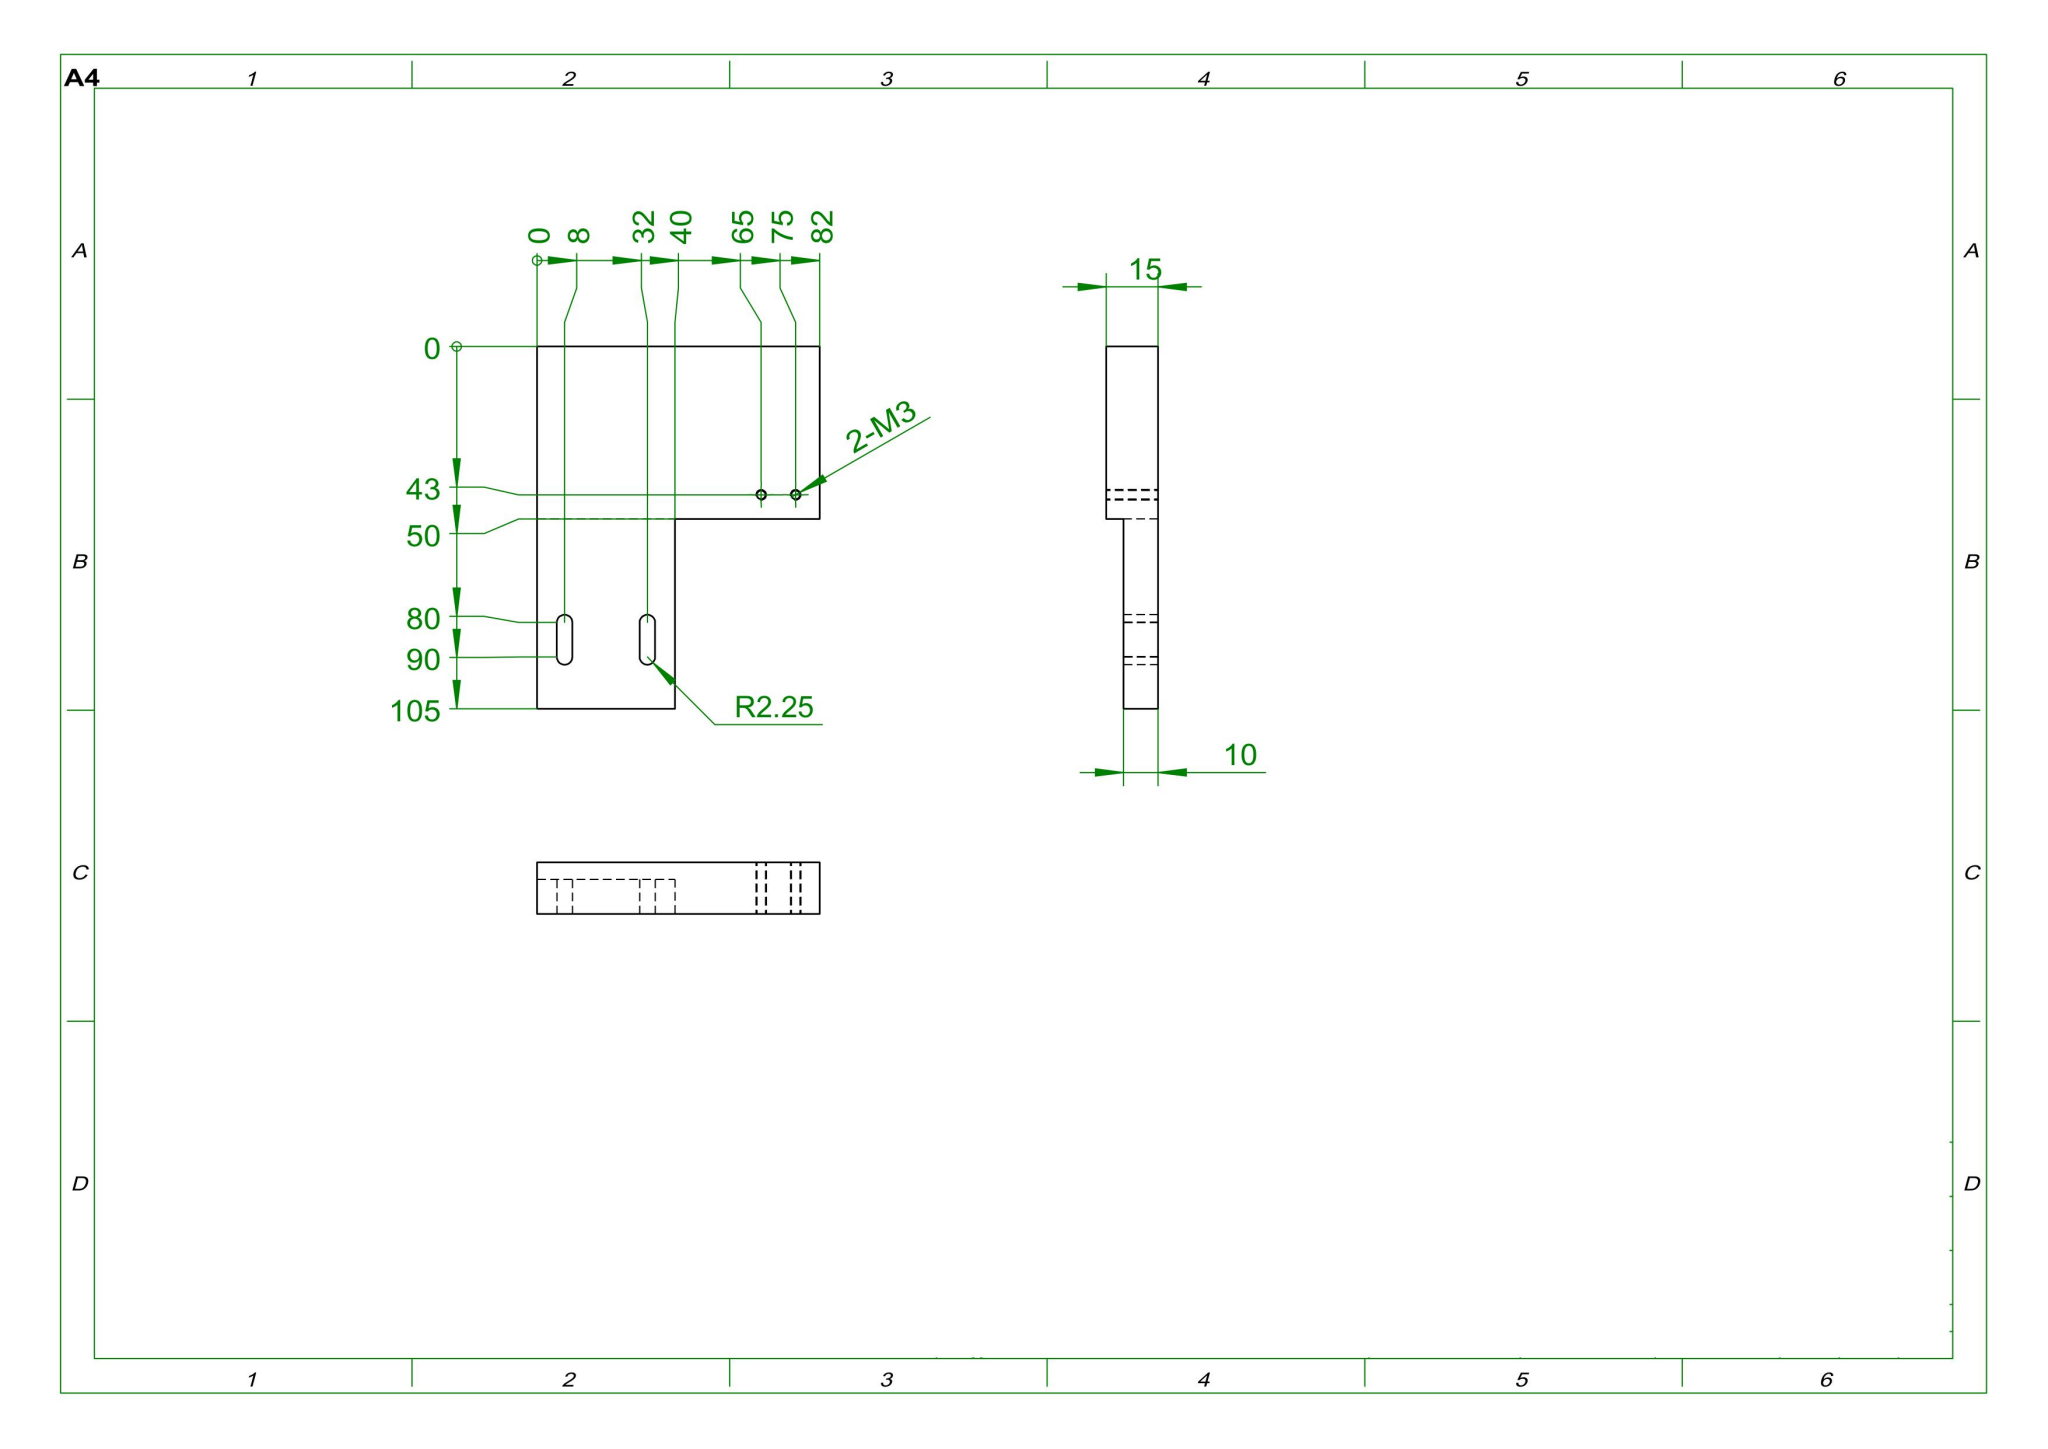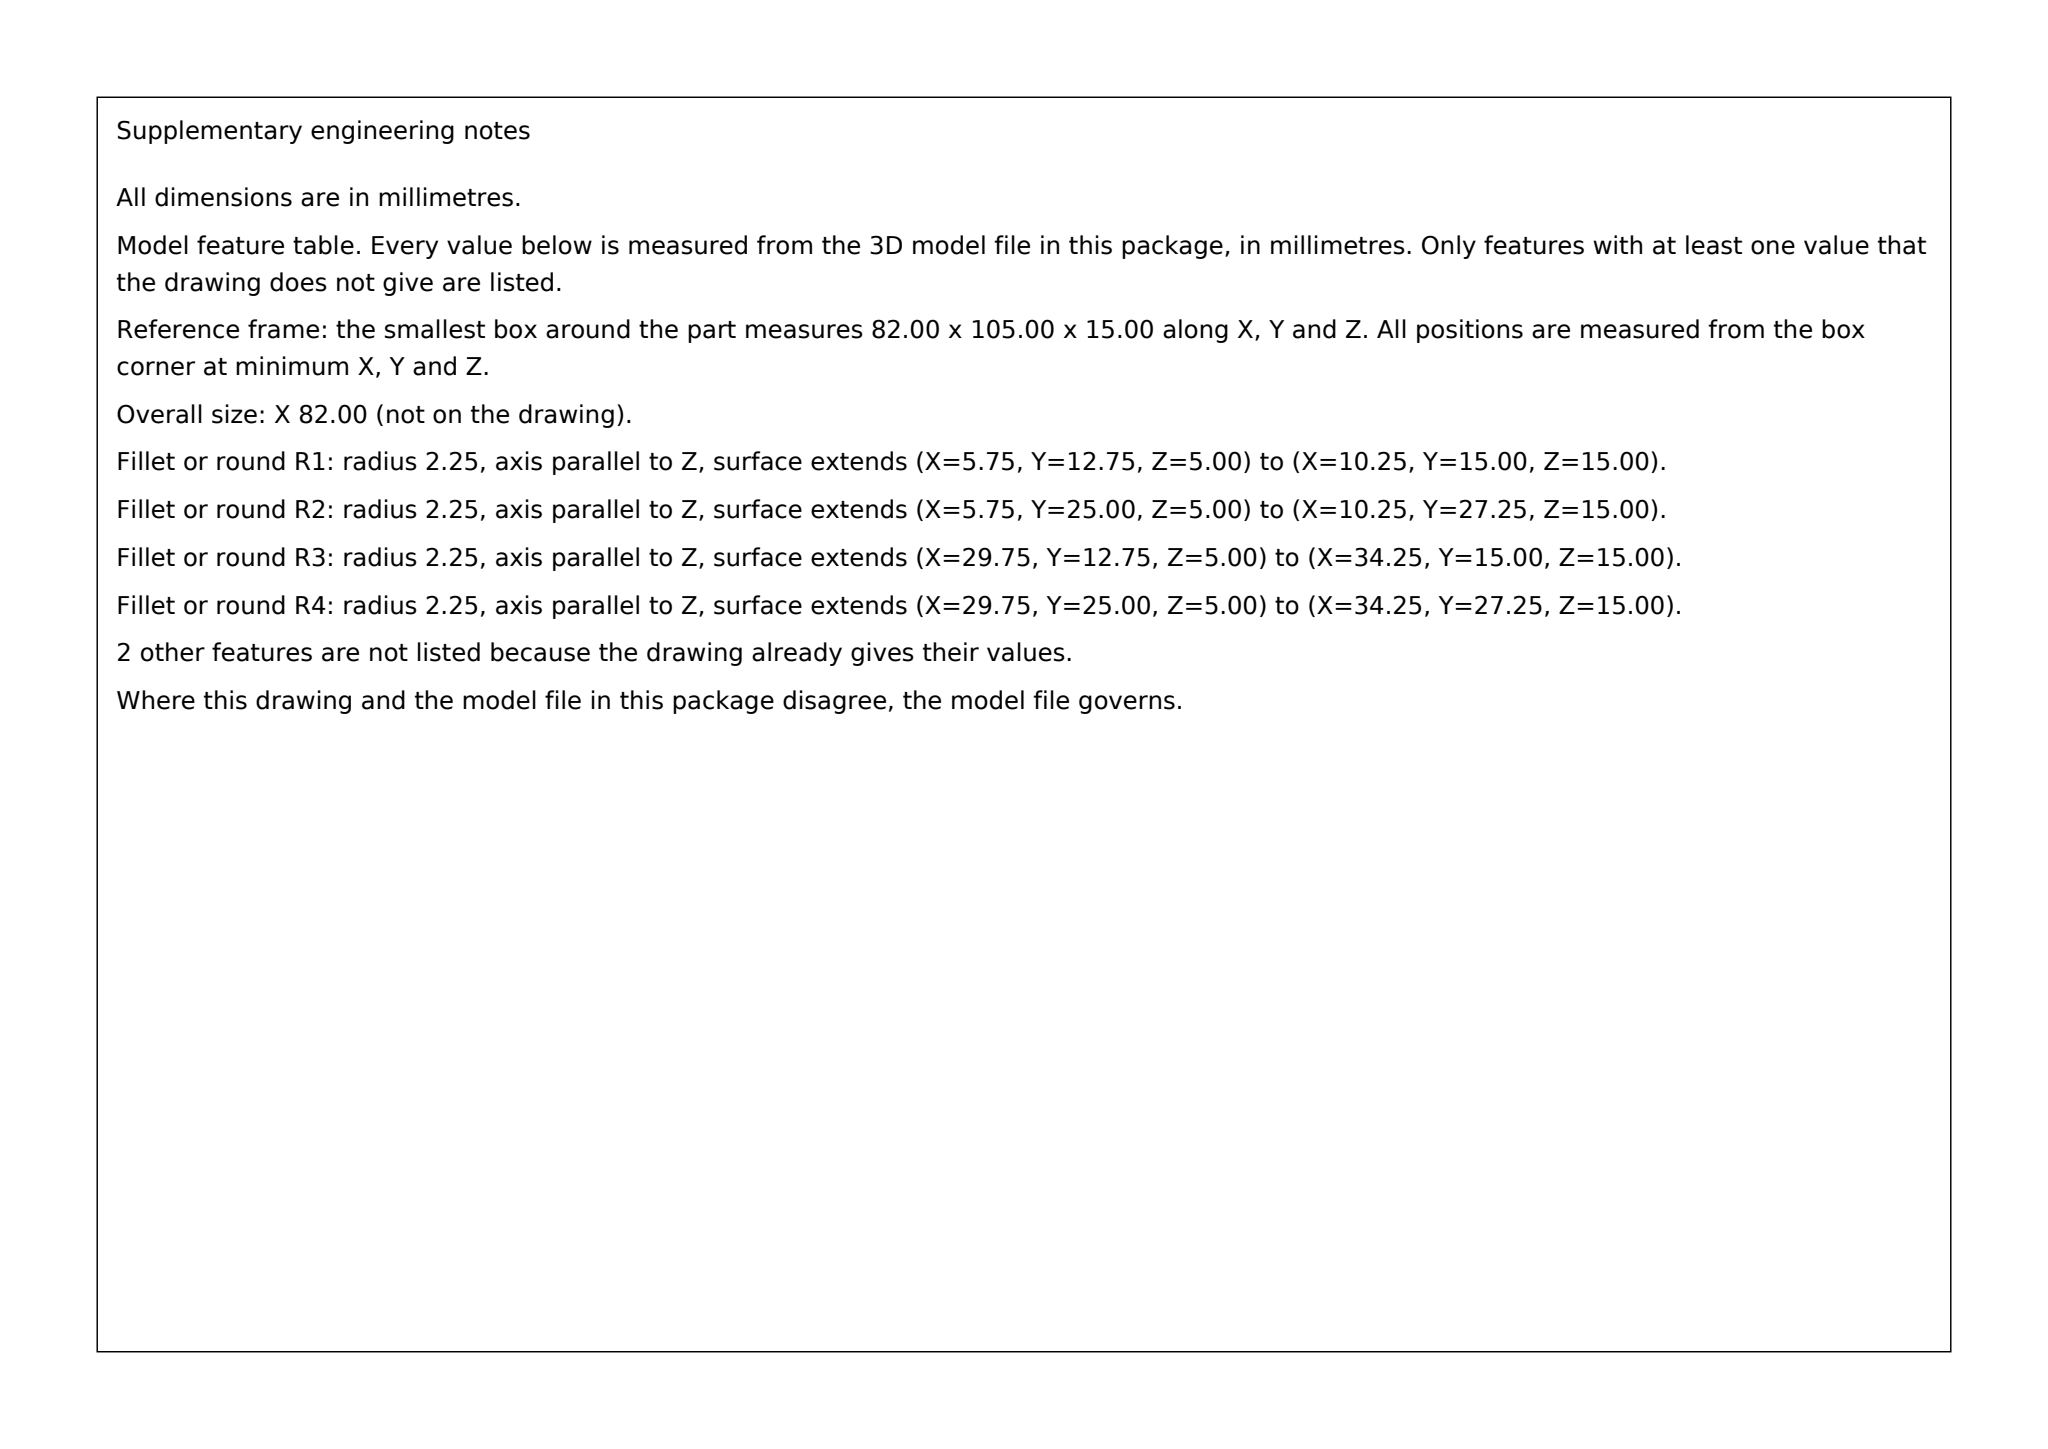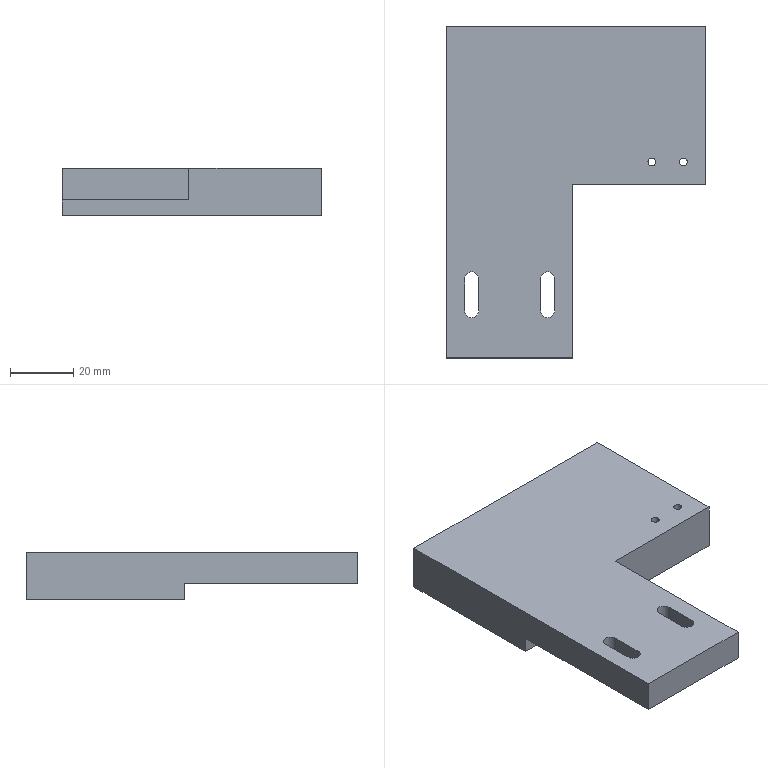Part | SolidWorks | mm | 1 solid | 21 faces | box 82 x 105 x 15 mm | volume 82135 mm3 | plane 13 | cylinder 8 | commonest cylinder face diameters 2.5 x4 4.5 x4
build123d program:
from build123d import *

# Parameters (mm, degrees)
BOSS_EXTRUDE1_DEPTH = 15
SKETCH2_W           = 40
SKETCH2_H           = 55
CUT_EXTRUDE1_DEPTH  = 5
CUT_EXTRUDE2_DEPTH  = 10
M3_TAPPED_HOLE1_D   = 2.5


with BuildPart() as part:
    # Sketch1 → Boss-Extrude1 (new body)
    with BuildSketch(Plane.XY):
        Polygon((40, 0), (40, 55), (82, 55), (82, 105), (0, 105), (0, 0), align=None)
    extrude(amount=BOSS_EXTRUDE1_DEPTH)

    # Sketch2 → Cut-Extrude1 (cut)
    with BuildSketch(Plane(origin=(0, 0, 0), x_dir=(-1, 0, 0), z_dir=(0, 0, -1))):
        with Locations((-20, 27.5)):
            Rectangle(SKETCH2_W, SKETCH2_H)
    extrude(amount=-CUT_EXTRUDE1_DEPTH, mode=Mode.SUBTRACT)

    # Sketch3 → Cut-Extrude2 (cut)
    with BuildSketch(Plane.XY.offset(15)):
        with BuildLine():
            Line((5.75, 15), (5.75, 25))
            ThreePointArc((5.75, 25), (8, 27.25), (10.25, 25))
            Line((10.25, 25), (10.25, 15))
            ThreePointArc((10.25, 15), (8, 12.75), (5.75, 15))
        make_face()
        with BuildLine():
            Line((34.25, 15), (34.25, 25))
            ThreePointArc((34.25, 25), (32, 27.25), (29.75, 25))
            Line((29.75, 25), (29.75, 15))
            ThreePointArc((29.75, 15), (32, 12.75), (34.25, 15))
        make_face()
    extrude(amount=-CUT_EXTRUDE2_DEPTH, mode=Mode.SUBTRACT)

    # M3 Tapped Hole1 (through all)
    with Locations(Plane(origin=(0, 0, 0), x_dir=(-1, 0, 0), z_dir=(0, 0, -1))):
        with Locations((-75, 62), (-65, 62)):
            Hole(M3_TAPPED_HOLE1_D / 2)


solid = part.part
STEP:
#1=CARTESIAN_POINT('',(76.25,62.,15.));
#2=VERTEX_POINT('',#1);
#3=CARTESIAN_POINT('',(73.75,62.,15.));
#4=VERTEX_POINT('',#3);
#5=CARTESIAN_POINT('',(75.,62.,15.));
#6=DIRECTION('',(0.,0.,-1.));
#7=DIRECTION('',(-1.,0.,0.));
#8=AXIS2_PLACEMENT_3D('',#5,#6,#7);
#9=CIRCLE('',#8,1.25);
#10=EDGE_CURVE('',#2,#4,#9,.T.);
#11=ORIENTED_EDGE('',*,*,#10,.F.);
#12=CARTESIAN_POINT('',(76.25,62.,-0.));
#13=VERTEX_POINT('',#12);
#14=CARTESIAN_POINT('',(76.25,62.,0.));
#15=DIRECTION('',(0.,0.,-1.));
#16=VECTOR('',#15,1000.);
#17=LINE('',#14,#16);
#18=EDGE_CURVE('',#2,#13,#17,.T.);
#19=ORIENTED_EDGE('',*,*,#18,.T.);
#20=CARTESIAN_POINT('',(73.75,62.,-0.));
#21=VERTEX_POINT('',#20);
#22=CARTESIAN_POINT('',(75.,62.,-0.));
#23=DIRECTION('',(0.,0.,-1.));
#24=DIRECTION('',(-1.,0.,0.));
#25=AXIS2_PLACEMENT_3D('',#22,#23,#24);
#26=CIRCLE('',#25,1.25);
#27=EDGE_CURVE('',#13,#21,#26,.T.);
#28=ORIENTED_EDGE('',*,*,#27,.T.);
#29=CARTESIAN_POINT('',(73.75,62.,0.));
#30=DIRECTION('',(0.,0.,-1.));
#31=VECTOR('',#30,1000.);
#32=LINE('',#29,#31);
#33=EDGE_CURVE('',#4,#21,#32,.T.);
#34=ORIENTED_EDGE('',*,*,#33,.F.);
#35=EDGE_LOOP('',(#11,#19,#28,#34));
#36=FACE_OUTER_BOUND('',#35,.T.);
#37=CARTESIAN_POINT('',(75.,62.,0.));
#38=DIRECTION('',(0.,0.,-1.));
#39=DIRECTION('',(-1.,0.,0.));
#40=AXIS2_PLACEMENT_3D('',#37,#38,#39);
#41=CYLINDRICAL_SURFACE('',#40,1.25);
#42=ADVANCED_FACE('',(#36),#41,.F.);
#43=CARTESIAN_POINT('',(66.25,62.,15.));
#44=VERTEX_POINT('',#43);
#45=CARTESIAN_POINT('',(63.75,62.,15.));
#46=VERTEX_POINT('',#45);
#47=CARTESIAN_POINT('',(65.,62.,15.));
#48=DIRECTION('',(0.,0.,-1.));
#49=DIRECTION('',(-1.,0.,0.));
#50=AXIS2_PLACEMENT_3D('',#47,#48,#49);
#51=CIRCLE('',#50,1.25);
#52=EDGE_CURVE('',#44,#46,#51,.T.);
#53=ORIENTED_EDGE('',*,*,#52,.F.);
#54=CARTESIAN_POINT('',(66.25,62.,-0.));
#55=VERTEX_POINT('',#54);
#56=CARTESIAN_POINT('',(66.25,62.,0.));
#57=DIRECTION('',(0.,0.,-1.));
#58=VECTOR('',#57,1000.);
#59=LINE('',#56,#58);
#60=EDGE_CURVE('',#44,#55,#59,.T.);
#61=ORIENTED_EDGE('',*,*,#60,.T.);
#62=CARTESIAN_POINT('',(63.75,62.,-0.));
#63=VERTEX_POINT('',#62);
#64=CARTESIAN_POINT('',(65.,62.,-0.));
#65=DIRECTION('',(0.,0.,-1.));
#66=DIRECTION('',(-1.,0.,0.));
#67=AXIS2_PLACEMENT_3D('',#64,#65,#66);
#68=CIRCLE('',#67,1.25);
#69=EDGE_CURVE('',#55,#63,#68,.T.);
#70=ORIENTED_EDGE('',*,*,#69,.T.);
#71=CARTESIAN_POINT('',(63.75,62.,0.));
#72=DIRECTION('',(0.,0.,-1.));
#73=VECTOR('',#72,1000.);
#74=LINE('',#71,#73);
#75=EDGE_CURVE('',#46,#63,#74,.T.);
#76=ORIENTED_EDGE('',*,*,#75,.F.);
#77=EDGE_LOOP('',(#53,#61,#70,#76));
#78=FACE_OUTER_BOUND('',#77,.T.);
#79=CARTESIAN_POINT('',(65.,62.,0.));
#80=DIRECTION('',(0.,0.,-1.));
#81=DIRECTION('',(-1.,0.,0.));
#82=AXIS2_PLACEMENT_3D('',#79,#80,#81);
#83=CYLINDRICAL_SURFACE('',#82,1.25);
#84=ADVANCED_FACE('',(#78),#83,.F.);
#85=CARTESIAN_POINT('',(40.,0.,5.));
#86=VERTEX_POINT('',#85);
#87=CARTESIAN_POINT('',(0.,0.,5.));
#88=VERTEX_POINT('',#87);
#89=CARTESIAN_POINT('',(40.,0.,5.));
#90=DIRECTION('',(-1.,0.,0.));
#91=VECTOR('',#90,1000.);
#92=LINE('',#89,#91);
#93=EDGE_CURVE('',#86,#88,#92,.T.);
#94=ORIENTED_EDGE('',*,*,#93,.F.);
#95=CARTESIAN_POINT('',(40.,0.,15.));
#96=VERTEX_POINT('',#95);
#97=CARTESIAN_POINT('',(40.,0.,15.));
#98=DIRECTION('',(0.,0.,-1.));
#99=VECTOR('',#98,1000.);
#100=LINE('',#97,#99);
#101=EDGE_CURVE('',#96,#86,#100,.T.);
#102=ORIENTED_EDGE('',*,*,#101,.F.);
#103=CARTESIAN_POINT('',(0.,0.,15.));
#104=VERTEX_POINT('',#103);
#105=CARTESIAN_POINT('',(0.,0.,15.));
#106=DIRECTION('',(1.,0.,0.));
#107=VECTOR('',#106,1000.);
#108=LINE('',#105,#107);
#109=EDGE_CURVE('',#104,#96,#108,.T.);
#110=ORIENTED_EDGE('',*,*,#109,.F.);
#111=CARTESIAN_POINT('',(0.,0.,15.));
#112=DIRECTION('',(0.,0.,-1.));
#113=VECTOR('',#112,1000.);
#114=LINE('',#111,#113);
#115=EDGE_CURVE('',#104,#88,#114,.T.);
#116=ORIENTED_EDGE('',*,*,#115,.T.);
#117=EDGE_LOOP('',(#94,#102,#110,#116));
#118=FACE_OUTER_BOUND('',#117,.T.);
#119=CARTESIAN_POINT('',(0.,0.,15.));
#120=DIRECTION('',(0.,1.,0.));
#121=DIRECTION('',(0.,0.,1.));
#122=AXIS2_PLACEMENT_3D('',#119,#120,#121);
#123=PLANE('',#122);
#124=ADVANCED_FACE('',(#118),#123,.F.);
#125=CARTESIAN_POINT('',(40.,55.,5.));
#126=VERTEX_POINT('',#125);
#127=CARTESIAN_POINT('',(40.,55.,5.));
#128=DIRECTION('',(0.,-1.,0.));
#129=VECTOR('',#128,1000.);
#130=LINE('',#127,#129);
#131=EDGE_CURVE('',#126,#86,#130,.T.);
#132=ORIENTED_EDGE('',*,*,#131,.F.);
#133=CARTESIAN_POINT('',(40.,55.,15.));
#134=VERTEX_POINT('',#133);
#135=CARTESIAN_POINT('',(40.,55.,15.));
#136=DIRECTION('',(0.,0.,-1.));
#137=VECTOR('',#136,1000.);
#138=LINE('',#135,#137);
#139=EDGE_CURVE('',#134,#126,#138,.T.);
#140=ORIENTED_EDGE('',*,*,#139,.F.);
#141=CARTESIAN_POINT('',(40.,0.,15.));
#142=DIRECTION('',(-0.,1.,0.));
#143=VECTOR('',#142,1000.);
#144=LINE('',#141,#143);
#145=EDGE_CURVE('',#96,#134,#144,.T.);
#146=ORIENTED_EDGE('',*,*,#145,.F.);
#147=ORIENTED_EDGE('',*,*,#101,.T.);
#148=EDGE_LOOP('',(#132,#140,#146,#147));
#149=FACE_OUTER_BOUND('',#148,.T.);
#150=CARTESIAN_POINT('',(40.,0.,15.));
#151=DIRECTION('',(-1.,-0.,0.));
#152=DIRECTION('',(0.,-1.,0.));
#153=AXIS2_PLACEMENT_3D('',#150,#151,#152);
#154=PLANE('',#153);
#155=ADVANCED_FACE('',(#149),#154,.F.);
#156=CARTESIAN_POINT('',(0.,105.,0.));
#157=VERTEX_POINT('',#156);
#158=CARTESIAN_POINT('',(0.,55.,0.));
#159=VERTEX_POINT('',#158);
#160=CARTESIAN_POINT('',(0.,0.,0.));
#161=DIRECTION('',(0.,-1.,0.));
#162=VECTOR('',#161,1000.);
#163=LINE('',#160,#162);
#164=EDGE_CURVE('',#157,#159,#163,.T.);
#165=ORIENTED_EDGE('',*,*,#164,.T.);
#166=CARTESIAN_POINT('',(-0.,55.,5.));
#167=VERTEX_POINT('',#166);
#168=CARTESIAN_POINT('',(-0.,55.,5.));
#169=DIRECTION('',(0.,0.,-1.));
#170=VECTOR('',#169,1000.);
#171=LINE('',#168,#170);
#172=EDGE_CURVE('',#167,#159,#171,.T.);
#173=ORIENTED_EDGE('',*,*,#172,.F.);
#174=CARTESIAN_POINT('',(-0.,55.,5.));
#175=DIRECTION('',(-0.,1.,0.));
#176=VECTOR('',#175,1000.);
#177=LINE('',#174,#176);
#178=EDGE_CURVE('',#88,#167,#177,.T.);
#179=ORIENTED_EDGE('',*,*,#178,.F.);
#180=ORIENTED_EDGE('',*,*,#115,.F.);
#181=CARTESIAN_POINT('',(0.,105.,15.));
#182=VERTEX_POINT('',#181);
#183=CARTESIAN_POINT('',(0.,0.,15.));
#184=DIRECTION('',(0.,-1.,0.));
#185=VECTOR('',#184,1000.);
#186=LINE('',#183,#185);
#187=EDGE_CURVE('',#182,#104,#186,.T.);
#188=ORIENTED_EDGE('',*,*,#187,.F.);
#189=CARTESIAN_POINT('',(0.,105.,15.));
#190=DIRECTION('',(0.,0.,-1.));
#191=VECTOR('',#190,1000.);
#192=LINE('',#189,#191);
#193=EDGE_CURVE('',#182,#157,#192,.T.);
#194=ORIENTED_EDGE('',*,*,#193,.T.);
#195=EDGE_LOOP('',(#165,#173,#179,#180,#188,#194));
#196=FACE_OUTER_BOUND('',#195,.T.);
#197=CARTESIAN_POINT('',(0.,0.,15.));
#198=DIRECTION('',(1.,0.,0.));
#199=DIRECTION('',(0.,0.,-1.));
#200=AXIS2_PLACEMENT_3D('',#197,#198,#199);
#201=PLANE('',#200);
#202=ADVANCED_FACE('',(#196),#201,.F.);
#203=CARTESIAN_POINT('',(82.,55.,0.));
#204=VERTEX_POINT('',#203);
#205=CARTESIAN_POINT('',(40.,55.,0.));
#206=DIRECTION('',(1.,0.,0.));
#207=VECTOR('',#206,1000.);
#208=LINE('',#205,#207);
#209=EDGE_CURVE('',#159,#204,#208,.T.);
#210=ORIENTED_EDGE('',*,*,#209,.T.);
#211=CARTESIAN_POINT('',(82.,55.,15.));
#212=VERTEX_POINT('',#211);
#213=CARTESIAN_POINT('',(82.,55.,15.));
#214=DIRECTION('',(0.,0.,-1.));
#215=VECTOR('',#214,1000.);
#216=LINE('',#213,#215);
#217=EDGE_CURVE('',#212,#204,#216,.T.);
#218=ORIENTED_EDGE('',*,*,#217,.F.);
#219=CARTESIAN_POINT('',(40.,55.,15.));
#220=DIRECTION('',(1.,0.,0.));
#221=VECTOR('',#220,1000.);
#222=LINE('',#219,#221);
#223=EDGE_CURVE('',#134,#212,#222,.T.);
#224=ORIENTED_EDGE('',*,*,#223,.F.);
#225=ORIENTED_EDGE('',*,*,#139,.T.);
#226=CARTESIAN_POINT('',(40.,55.,5.));
#227=DIRECTION('',(1.,0.,0.));
#228=VECTOR('',#227,1000.);
#229=LINE('',#226,#228);
#230=EDGE_CURVE('',#167,#126,#229,.T.);
#231=ORIENTED_EDGE('',*,*,#230,.F.);
#232=ORIENTED_EDGE('',*,*,#172,.T.);
#233=EDGE_LOOP('',(#210,#218,#224,#225,#231,#232));
#234=FACE_OUTER_BOUND('',#233,.T.);
#235=CARTESIAN_POINT('',(40.,55.,15.));
#236=DIRECTION('',(0.,1.,0.));
#237=DIRECTION('',(0.,0.,1.));
#238=AXIS2_PLACEMENT_3D('',#235,#236,#237);
#239=PLANE('',#238);
#240=ADVANCED_FACE('',(#234),#239,.F.);
#241=CARTESIAN_POINT('',(82.,105.,0.));
#242=VERTEX_POINT('',#241);
#243=CARTESIAN_POINT('',(82.,55.,0.));
#244=DIRECTION('',(0.,1.,0.));
#245=VECTOR('',#244,1000.);
#246=LINE('',#243,#245);
#247=EDGE_CURVE('',#204,#242,#246,.T.);
#248=ORIENTED_EDGE('',*,*,#247,.T.);
#249=CARTESIAN_POINT('',(82.,105.,15.));
#250=VERTEX_POINT('',#249);
#251=CARTESIAN_POINT('',(82.,105.,15.));
#252=DIRECTION('',(0.,0.,-1.));
#253=VECTOR('',#252,1000.);
#254=LINE('',#251,#253);
#255=EDGE_CURVE('',#250,#242,#254,.T.);
#256=ORIENTED_EDGE('',*,*,#255,.F.);
#257=CARTESIAN_POINT('',(82.,55.,15.));
#258=DIRECTION('',(0.,1.,0.));
#259=VECTOR('',#258,1000.);
#260=LINE('',#257,#259);
#261=EDGE_CURVE('',#212,#250,#260,.T.);
#262=ORIENTED_EDGE('',*,*,#261,.F.);
#263=ORIENTED_EDGE('',*,*,#217,.T.);
#264=EDGE_LOOP('',(#248,#256,#262,#263));
#265=FACE_OUTER_BOUND('',#264,.T.);
#266=CARTESIAN_POINT('',(82.,55.,15.));
#267=DIRECTION('',(-1.,0.,0.));
#268=DIRECTION('',(0.,0.,1.));
#269=AXIS2_PLACEMENT_3D('',#266,#267,#268);
#270=PLANE('',#269);
#271=ADVANCED_FACE('',(#265),#270,.F.);
#272=CARTESIAN_POINT('',(0.,105.,0.));
#273=DIRECTION('',(-1.,0.,0.));
#274=VECTOR('',#273,1000.);
#275=LINE('',#272,#274);
#276=EDGE_CURVE('',#242,#157,#275,.T.);
#277=ORIENTED_EDGE('',*,*,#276,.T.);
#278=ORIENTED_EDGE('',*,*,#193,.F.);
#279=CARTESIAN_POINT('',(0.,105.,15.));
#280=DIRECTION('',(-1.,0.,0.));
#281=VECTOR('',#280,1000.);
#282=LINE('',#279,#281);
#283=EDGE_CURVE('',#250,#182,#282,.T.);
#284=ORIENTED_EDGE('',*,*,#283,.F.);
#285=ORIENTED_EDGE('',*,*,#255,.T.);
#286=EDGE_LOOP('',(#277,#278,#284,#285));
#287=FACE_OUTER_BOUND('',#286,.T.);
#288=CARTESIAN_POINT('',(0.,105.,15.));
#289=DIRECTION('',(0.,-1.,0.));
#290=DIRECTION('',(0.,0.,-1.));
#291=AXIS2_PLACEMENT_3D('',#288,#289,#290);
#292=PLANE('',#291);
#293=ADVANCED_FACE('',(#287),#292,.F.);
#294=CARTESIAN_POINT('',(75.,62.,15.));
#295=DIRECTION('',(0.,0.,-1.));
#296=DIRECTION('',(-1.,0.,0.));
#297=AXIS2_PLACEMENT_3D('',#294,#295,#296);
#298=CIRCLE('',#297,1.25);
#299=EDGE_CURVE('',#4,#2,#298,.T.);
#300=ORIENTED_EDGE('',*,*,#299,.T.);
#301=ORIENTED_EDGE('',*,*,#10,.T.);
#302=EDGE_LOOP('',(#300,#301));
#303=FACE_BOUND('',#302,.T.);
#304=CARTESIAN_POINT('',(65.,62.,15.));
#305=DIRECTION('',(0.,0.,-1.));
#306=DIRECTION('',(-1.,0.,0.));
#307=AXIS2_PLACEMENT_3D('',#304,#305,#306);
#308=CIRCLE('',#307,1.25);
#309=EDGE_CURVE('',#46,#44,#308,.T.);
#310=ORIENTED_EDGE('',*,*,#309,.T.);
#311=ORIENTED_EDGE('',*,*,#52,.T.);
#312=EDGE_LOOP('',(#310,#311));
#313=FACE_BOUND('',#312,.T.);
#314=CARTESIAN_POINT('',(34.25,15.,15.));
#315=VERTEX_POINT('',#314);
#316=CARTESIAN_POINT('',(34.25,25.,15.));
#317=VERTEX_POINT('',#316);
#318=CARTESIAN_POINT('',(34.25,15.,15.));
#319=DIRECTION('',(0.,1.,0.));
#320=VECTOR('',#319,1000.);
#321=LINE('',#318,#320);
#322=EDGE_CURVE('',#315,#317,#321,.T.);
#323=ORIENTED_EDGE('',*,*,#322,.F.);
#324=CARTESIAN_POINT('',(29.75,15.,15.));
#325=VERTEX_POINT('',#324);
#326=CARTESIAN_POINT('',(32.,15.,15.));
#327=DIRECTION('',(0.,0.,1.));
#328=DIRECTION('',(-1.,0.,0.));
#329=AXIS2_PLACEMENT_3D('',#326,#327,#328);
#330=CIRCLE('',#329,2.25);
#331=EDGE_CURVE('',#325,#315,#330,.T.);
#332=ORIENTED_EDGE('',*,*,#331,.F.);
#333=CARTESIAN_POINT('',(29.75,25.,15.));
#334=VERTEX_POINT('',#333);
#335=CARTESIAN_POINT('',(29.75,15.,15.));
#336=DIRECTION('',(0.,-1.,0.));
#337=VECTOR('',#336,1000.);
#338=LINE('',#335,#337);
#339=EDGE_CURVE('',#334,#325,#338,.T.);
#340=ORIENTED_EDGE('',*,*,#339,.F.);
#341=CARTESIAN_POINT('',(32.,25.,15.));
#342=DIRECTION('',(0.,0.,1.));
#343=DIRECTION('',(-1.,0.,0.));
#344=AXIS2_PLACEMENT_3D('',#341,#342,#343);
#345=CIRCLE('',#344,2.25);
#346=EDGE_CURVE('',#317,#334,#345,.T.);
#347=ORIENTED_EDGE('',*,*,#346,.F.);
#348=EDGE_LOOP('',(#323,#332,#340,#347));
#349=FACE_BOUND('',#348,.T.);
#350=CARTESIAN_POINT('',(10.25,15.,15.));
#351=VERTEX_POINT('',#350);
#352=CARTESIAN_POINT('',(10.25,25.,15.));
#353=VERTEX_POINT('',#352);
#354=CARTESIAN_POINT('',(10.25,15.,15.));
#355=DIRECTION('',(-0.,1.,0.));
#356=VECTOR('',#355,1000.);
#357=LINE('',#354,#356);
#358=EDGE_CURVE('',#351,#353,#357,.T.);
#359=ORIENTED_EDGE('',*,*,#358,.F.);
#360=CARTESIAN_POINT('',(5.75,15.,15.));
#361=VERTEX_POINT('',#360);
#362=CARTESIAN_POINT('',(8.,15.,15.));
#363=DIRECTION('',(0.,0.,1.));
#364=DIRECTION('',(1.,0.,0.));
#365=AXIS2_PLACEMENT_3D('',#362,#363,#364);
#366=CIRCLE('',#365,2.25);
#367=EDGE_CURVE('',#361,#351,#366,.T.);
#368=ORIENTED_EDGE('',*,*,#367,.F.);
#369=CARTESIAN_POINT('',(5.75,25.,15.));
#370=VERTEX_POINT('',#369);
#371=CARTESIAN_POINT('',(5.75,15.,15.));
#372=DIRECTION('',(0.,-1.,0.));
#373=VECTOR('',#372,1000.);
#374=LINE('',#371,#373);
#375=EDGE_CURVE('',#370,#361,#374,.T.);
#376=ORIENTED_EDGE('',*,*,#375,.F.);
#377=CARTESIAN_POINT('',(8.,25.,15.));
#378=DIRECTION('',(0.,0.,1.));
#379=DIRECTION('',(1.,0.,0.));
#380=AXIS2_PLACEMENT_3D('',#377,#378,#379);
#381=CIRCLE('',#380,2.25);
#382=EDGE_CURVE('',#353,#370,#381,.T.);
#383=ORIENTED_EDGE('',*,*,#382,.F.);
#384=EDGE_LOOP('',(#359,#368,#376,#383));
#385=FACE_BOUND('',#384,.T.);
#386=ORIENTED_EDGE('',*,*,#187,.T.);
#387=ORIENTED_EDGE('',*,*,#109,.T.);
#388=ORIENTED_EDGE('',*,*,#145,.T.);
#389=ORIENTED_EDGE('',*,*,#223,.T.);
#390=ORIENTED_EDGE('',*,*,#261,.T.);
#391=ORIENTED_EDGE('',*,*,#283,.T.);
#392=EDGE_LOOP('',(#386,#387,#388,#389,#390,#391));
#393=FACE_OUTER_BOUND('',#392,.T.);
#394=CARTESIAN_POINT('',(0.,0.,15.));
#395=DIRECTION('',(0.,0.,-1.));
#396=DIRECTION('',(-1.,0.,0.));
#397=AXIS2_PLACEMENT_3D('',#394,#395,#396);
#398=PLANE('',#397);
#399=ADVANCED_FACE('',(#303,#313,#349,#385,#393),#398,.F.);
#400=CARTESIAN_POINT('',(75.,62.,-0.));
#401=DIRECTION('',(0.,0.,-1.));
#402=DIRECTION('',(-1.,0.,0.));
#403=AXIS2_PLACEMENT_3D('',#400,#401,#402);
#404=CIRCLE('',#403,1.25);
#405=EDGE_CURVE('',#21,#13,#404,.T.);
#406=ORIENTED_EDGE('',*,*,#405,.F.);
#407=ORIENTED_EDGE('',*,*,#27,.F.);
#408=EDGE_LOOP('',(#406,#407));
#409=FACE_BOUND('',#408,.T.);
#410=CARTESIAN_POINT('',(65.,62.,-0.));
#411=DIRECTION('',(0.,0.,-1.));
#412=DIRECTION('',(-1.,0.,0.));
#413=AXIS2_PLACEMENT_3D('',#410,#411,#412);
#414=CIRCLE('',#413,1.25);
#415=EDGE_CURVE('',#63,#55,#414,.T.);
#416=ORIENTED_EDGE('',*,*,#415,.F.);
#417=ORIENTED_EDGE('',*,*,#69,.F.);
#418=EDGE_LOOP('',(#416,#417));
#419=FACE_BOUND('',#418,.T.);
#420=ORIENTED_EDGE('',*,*,#209,.F.);
#421=ORIENTED_EDGE('',*,*,#164,.F.);
#422=ORIENTED_EDGE('',*,*,#276,.F.);
#423=ORIENTED_EDGE('',*,*,#247,.F.);
#424=EDGE_LOOP('',(#420,#421,#422,#423));
#425=FACE_OUTER_BOUND('',#424,.T.);
#426=CARTESIAN_POINT('',(0.,0.,0.));
#427=DIRECTION('',(0.,0.,-1.));
#428=DIRECTION('',(-1.,0.,0.));
#429=AXIS2_PLACEMENT_3D('',#426,#427,#428);
#430=PLANE('',#429);
#431=ADVANCED_FACE('',(#409,#419,#425),#430,.T.);
#432=CARTESIAN_POINT('',(29.75,15.,5.));
#433=VERTEX_POINT('',#432);
#434=CARTESIAN_POINT('',(34.25,15.,5.));
#435=VERTEX_POINT('',#434);
#436=CARTESIAN_POINT('',(32.,15.,5.));
#437=DIRECTION('',(0.,0.,1.));
#438=DIRECTION('',(-1.,0.,0.));
#439=AXIS2_PLACEMENT_3D('',#436,#437,#438);
#440=CIRCLE('',#439,2.25);
#441=EDGE_CURVE('',#433,#435,#440,.T.);
#442=ORIENTED_EDGE('',*,*,#441,.T.);
#443=CARTESIAN_POINT('',(34.25,25.,5.));
#444=VERTEX_POINT('',#443);
#445=CARTESIAN_POINT('',(34.25,15.,5.));
#446=DIRECTION('',(0.,1.,0.));
#447=VECTOR('',#446,1000.);
#448=LINE('',#445,#447);
#449=EDGE_CURVE('',#435,#444,#448,.T.);
#450=ORIENTED_EDGE('',*,*,#449,.T.);
#451=CARTESIAN_POINT('',(29.75,25.,5.));
#452=VERTEX_POINT('',#451);
#453=CARTESIAN_POINT('',(32.,25.,5.));
#454=DIRECTION('',(0.,0.,1.));
#455=DIRECTION('',(-1.,0.,0.));
#456=AXIS2_PLACEMENT_3D('',#453,#454,#455);
#457=CIRCLE('',#456,2.25);
#458=EDGE_CURVE('',#444,#452,#457,.T.);
#459=ORIENTED_EDGE('',*,*,#458,.T.);
#460=CARTESIAN_POINT('',(29.75,15.,5.));
#461=DIRECTION('',(0.,-1.,0.));
#462=VECTOR('',#461,1000.);
#463=LINE('',#460,#462);
#464=EDGE_CURVE('',#452,#433,#463,.T.);
#465=ORIENTED_EDGE('',*,*,#464,.T.);
#466=EDGE_LOOP('',(#442,#450,#459,#465));
#467=FACE_BOUND('',#466,.T.);
#468=CARTESIAN_POINT('',(5.75,15.,5.));
#469=VERTEX_POINT('',#468);
#470=CARTESIAN_POINT('',(10.25,15.,5.));
#471=VERTEX_POINT('',#470);
#472=CARTESIAN_POINT('',(8.,15.,5.));
#473=DIRECTION('',(0.,0.,1.));
#474=DIRECTION('',(1.,0.,0.));
#475=AXIS2_PLACEMENT_3D('',#472,#473,#474);
#476=CIRCLE('',#475,2.25);
#477=EDGE_CURVE('',#469,#471,#476,.T.);
#478=ORIENTED_EDGE('',*,*,#477,.T.);
#479=CARTESIAN_POINT('',(10.25,25.,5.));
#480=VERTEX_POINT('',#479);
#481=CARTESIAN_POINT('',(10.25,15.,5.));
#482=DIRECTION('',(-0.,1.,0.));
#483=VECTOR('',#482,1000.);
#484=LINE('',#481,#483);
#485=EDGE_CURVE('',#471,#480,#484,.T.);
#486=ORIENTED_EDGE('',*,*,#485,.T.);
#487=CARTESIAN_POINT('',(5.75,25.,5.));
#488=VERTEX_POINT('',#487);
#489=CARTESIAN_POINT('',(8.,25.,5.));
#490=DIRECTION('',(0.,0.,1.));
#491=DIRECTION('',(1.,0.,0.));
#492=AXIS2_PLACEMENT_3D('',#489,#490,#491);
#493=CIRCLE('',#492,2.25);
#494=EDGE_CURVE('',#480,#488,#493,.T.);
#495=ORIENTED_EDGE('',*,*,#494,.T.);
#496=CARTESIAN_POINT('',(5.75,15.,5.));
#497=DIRECTION('',(0.,-1.,0.));
#498=VECTOR('',#497,1000.);
#499=LINE('',#496,#498);
#500=EDGE_CURVE('',#488,#469,#499,.T.);
#501=ORIENTED_EDGE('',*,*,#500,.T.);
#502=EDGE_LOOP('',(#478,#486,#495,#501));
#503=FACE_BOUND('',#502,.T.);
#504=ORIENTED_EDGE('',*,*,#131,.T.);
#505=ORIENTED_EDGE('',*,*,#93,.T.);
#506=ORIENTED_EDGE('',*,*,#178,.T.);
#507=ORIENTED_EDGE('',*,*,#230,.T.);
#508=EDGE_LOOP('',(#504,#505,#506,#507));
#509=FACE_OUTER_BOUND('',#508,.T.);
#510=CARTESIAN_POINT('',(0.,0.,5.));
#511=DIRECTION('',(0.,0.,-1.));
#512=DIRECTION('',(-1.,0.,0.));
#513=AXIS2_PLACEMENT_3D('',#510,#511,#512);
#514=PLANE('',#513);
#515=ADVANCED_FACE('',(#467,#503,#509),#514,.T.);
#516=ORIENTED_EDGE('',*,*,#367,.T.);
#517=CARTESIAN_POINT('',(10.25,15.,5.));
#518=DIRECTION('',(0.,0.,1.));
#519=VECTOR('',#518,1000.);
#520=LINE('',#517,#519);
#521=EDGE_CURVE('',#471,#351,#520,.T.);
#522=ORIENTED_EDGE('',*,*,#521,.F.);
#523=ORIENTED_EDGE('',*,*,#477,.F.);
#524=CARTESIAN_POINT('',(5.75,15.,5.));
#525=DIRECTION('',(0.,0.,1.));
#526=VECTOR('',#525,1000.);
#527=LINE('',#524,#526);
#528=EDGE_CURVE('',#469,#361,#527,.T.);
#529=ORIENTED_EDGE('',*,*,#528,.T.);
#530=EDGE_LOOP('',(#516,#522,#523,#529));
#531=FACE_OUTER_BOUND('',#530,.T.);
#532=CARTESIAN_POINT('',(8.,15.,5.));
#533=DIRECTION('',(0.,0.,1.));
#534=DIRECTION('',(1.,0.,0.));
#535=AXIS2_PLACEMENT_3D('',#532,#533,#534);
#536=CYLINDRICAL_SURFACE('',#535,2.25);
#537=ADVANCED_FACE('',(#531),#536,.F.);
#538=ORIENTED_EDGE('',*,*,#375,.T.);
#539=ORIENTED_EDGE('',*,*,#528,.F.);
#540=ORIENTED_EDGE('',*,*,#500,.F.);
#541=CARTESIAN_POINT('',(5.75,25.,5.));
#542=DIRECTION('',(0.,0.,1.));
#543=VECTOR('',#542,1000.);
#544=LINE('',#541,#543);
#545=EDGE_CURVE('',#488,#370,#544,.T.);
#546=ORIENTED_EDGE('',*,*,#545,.T.);
#547=EDGE_LOOP('',(#538,#539,#540,#546));
#548=FACE_OUTER_BOUND('',#547,.T.);
#549=CARTESIAN_POINT('',(5.75,15.,5.));
#550=DIRECTION('',(-1.,-0.,0.));
#551=DIRECTION('',(0.,-1.,0.));
#552=AXIS2_PLACEMENT_3D('',#549,#550,#551);
#553=PLANE('',#552);
#554=ADVANCED_FACE('',(#548),#553,.F.);
#555=ORIENTED_EDGE('',*,*,#382,.T.);
#556=ORIENTED_EDGE('',*,*,#545,.F.);
#557=ORIENTED_EDGE('',*,*,#494,.F.);
#558=CARTESIAN_POINT('',(10.25,25.,5.));
#559=DIRECTION('',(0.,0.,1.));
#560=VECTOR('',#559,1000.);
#561=LINE('',#558,#560);
#562=EDGE_CURVE('',#480,#353,#561,.T.);
#563=ORIENTED_EDGE('',*,*,#562,.T.);
#564=EDGE_LOOP('',(#555,#556,#557,#563));
#565=FACE_OUTER_BOUND('',#564,.T.);
#566=CARTESIAN_POINT('',(8.,25.,5.));
#567=DIRECTION('',(0.,0.,1.));
#568=DIRECTION('',(1.,0.,0.));
#569=AXIS2_PLACEMENT_3D('',#566,#567,#568);
#570=CYLINDRICAL_SURFACE('',#569,2.25);
#571=ADVANCED_FACE('',(#565),#570,.F.);
#572=ORIENTED_EDGE('',*,*,#358,.T.);
#573=ORIENTED_EDGE('',*,*,#562,.F.);
#574=ORIENTED_EDGE('',*,*,#485,.F.);
#575=ORIENTED_EDGE('',*,*,#521,.T.);
#576=EDGE_LOOP('',(#572,#573,#574,#575));
#577=FACE_OUTER_BOUND('',#576,.T.);
#578=CARTESIAN_POINT('',(10.25,15.,5.));
#579=DIRECTION('',(1.,0.,0.));
#580=DIRECTION('',(-0.,1.,0.));
#581=AXIS2_PLACEMENT_3D('',#578,#579,#580);
#582=PLANE('',#581);
#583=ADVANCED_FACE('',(#577),#582,.F.);
#584=ORIENTED_EDGE('',*,*,#331,.T.);
#585=CARTESIAN_POINT('',(34.25,15.,5.));
#586=DIRECTION('',(0.,0.,1.));
#587=VECTOR('',#586,1000.);
#588=LINE('',#585,#587);
#589=EDGE_CURVE('',#435,#315,#588,.T.);
#590=ORIENTED_EDGE('',*,*,#589,.F.);
#591=ORIENTED_EDGE('',*,*,#441,.F.);
#592=CARTESIAN_POINT('',(29.75,15.,5.));
#593=DIRECTION('',(0.,0.,1.));
#594=VECTOR('',#593,1000.);
#595=LINE('',#592,#594);
#596=EDGE_CURVE('',#433,#325,#595,.T.);
#597=ORIENTED_EDGE('',*,*,#596,.T.);
#598=EDGE_LOOP('',(#584,#590,#591,#597));
#599=FACE_OUTER_BOUND('',#598,.T.);
#600=CARTESIAN_POINT('',(32.,15.,5.));
#601=DIRECTION('',(0.,0.,1.));
#602=DIRECTION('',(1.,0.,0.));
#603=AXIS2_PLACEMENT_3D('',#600,#601,#602);
#604=CYLINDRICAL_SURFACE('',#603,2.25);
#605=ADVANCED_FACE('',(#599),#604,.F.);
#606=ORIENTED_EDGE('',*,*,#339,.T.);
#607=ORIENTED_EDGE('',*,*,#596,.F.);
#608=ORIENTED_EDGE('',*,*,#464,.F.);
#609=CARTESIAN_POINT('',(29.75,25.,5.));
#610=DIRECTION('',(0.,0.,1.));
#611=VECTOR('',#610,1000.);
#612=LINE('',#609,#611);
#613=EDGE_CURVE('',#452,#334,#612,.T.);
#614=ORIENTED_EDGE('',*,*,#613,.T.);
#615=EDGE_LOOP('',(#606,#607,#608,#614));
#616=FACE_OUTER_BOUND('',#615,.T.);
#617=CARTESIAN_POINT('',(29.75,15.,5.));
#618=DIRECTION('',(-1.,-0.,0.));
#619=DIRECTION('',(0.,-1.,0.));
#620=AXIS2_PLACEMENT_3D('',#617,#618,#619);
#621=PLANE('',#620);
#622=ADVANCED_FACE('',(#616),#621,.F.);
#623=ORIENTED_EDGE('',*,*,#346,.T.);
#624=ORIENTED_EDGE('',*,*,#613,.F.);
#625=ORIENTED_EDGE('',*,*,#458,.F.);
#626=CARTESIAN_POINT('',(34.25,25.,5.));
#627=DIRECTION('',(0.,0.,1.));
#628=VECTOR('',#627,1000.);
#629=LINE('',#626,#628);
#630=EDGE_CURVE('',#444,#317,#629,.T.);
#631=ORIENTED_EDGE('',*,*,#630,.T.);
#632=EDGE_LOOP('',(#623,#624,#625,#631));
#633=FACE_OUTER_BOUND('',#632,.T.);
#634=CARTESIAN_POINT('',(32.,25.,5.));
#635=DIRECTION('',(0.,0.,1.));
#636=DIRECTION('',(1.,0.,0.));
#637=AXIS2_PLACEMENT_3D('',#634,#635,#636);
#638=CYLINDRICAL_SURFACE('',#637,2.25);
#639=ADVANCED_FACE('',(#633),#638,.F.);
#640=ORIENTED_EDGE('',*,*,#322,.T.);
#641=ORIENTED_EDGE('',*,*,#630,.F.);
#642=ORIENTED_EDGE('',*,*,#449,.F.);
#643=ORIENTED_EDGE('',*,*,#589,.T.);
#644=EDGE_LOOP('',(#640,#641,#642,#643));
#645=FACE_OUTER_BOUND('',#644,.T.);
#646=CARTESIAN_POINT('',(34.25,15.,5.));
#647=DIRECTION('',(1.,0.,0.));
#648=DIRECTION('',(0.,0.,-1.));
#649=AXIS2_PLACEMENT_3D('',#646,#647,#648);
#650=PLANE('',#649);
#651=ADVANCED_FACE('',(#645),#650,.F.);
#652=ORIENTED_EDGE('',*,*,#60,.F.);
#653=ORIENTED_EDGE('',*,*,#309,.F.);
#654=ORIENTED_EDGE('',*,*,#75,.T.);
#655=ORIENTED_EDGE('',*,*,#415,.T.);
#656=EDGE_LOOP('',(#652,#653,#654,#655));
#657=FACE_OUTER_BOUND('',#656,.T.);
#658=CARTESIAN_POINT('',(65.,62.,0.));
#659=DIRECTION('',(0.,0.,-1.));
#660=DIRECTION('',(-1.,0.,0.));
#661=AXIS2_PLACEMENT_3D('',#658,#659,#660);
#662=CYLINDRICAL_SURFACE('',#661,1.25);
#663=ADVANCED_FACE('',(#657),#662,.F.);
#664=ORIENTED_EDGE('',*,*,#18,.F.);
#665=ORIENTED_EDGE('',*,*,#299,.F.);
#666=ORIENTED_EDGE('',*,*,#33,.T.);
#667=ORIENTED_EDGE('',*,*,#405,.T.);
#668=EDGE_LOOP('',(#664,#665,#666,#667));
#669=FACE_OUTER_BOUND('',#668,.T.);
#670=CARTESIAN_POINT('',(75.,62.,0.));
#671=DIRECTION('',(0.,0.,-1.));
#672=DIRECTION('',(-1.,0.,0.));
#673=AXIS2_PLACEMENT_3D('',#670,#671,#672);
#674=CYLINDRICAL_SURFACE('',#673,1.25);
#675=ADVANCED_FACE('',(#669),#674,.F.);
#676=CLOSED_SHELL('',(#42,#84,#124,#155,#202,#240,#271,#293,#399,#431,#515,#537,#554,#571,#583,#605,#622,#639,#651,#663,#675));
#677=MANIFOLD_SOLID_BREP('',#676);
#678=CARTESIAN_POINT('',(0.,0.,0.));
#679=DIRECTION('',(0.,0.,1.));
#680=DIRECTION('',(1.,0.,0.));
#681=AXIS2_PLACEMENT_3D('',#678,#679,#680);
#682=(LENGTH_UNIT()NAMED_UNIT(*)SI_UNIT(.MILLI.,.METRE.));
#683=UNCERTAINTY_MEASURE_WITH_UNIT(LENGTH_MEASURE(0.00001),#682,'','');
#684=(NAMED_UNIT(*)PLANE_ANGLE_UNIT()SI_UNIT($,.RADIAN.));
#685=(NAMED_UNIT(*)SI_UNIT($,.STERADIAN.)SOLID_ANGLE_UNIT());
#686=(GEOMETRIC_REPRESENTATION_CONTEXT(3)GLOBAL_UNCERTAINTY_ASSIGNED_CONTEXT((#683))GLOBAL_UNIT_ASSIGNED_CONTEXT((#682,#684,#685))REPRESENTATION_CONTEXT('',''));
#687=ADVANCED_BREP_SHAPE_REPRESENTATION('',(#677,#681),#686);